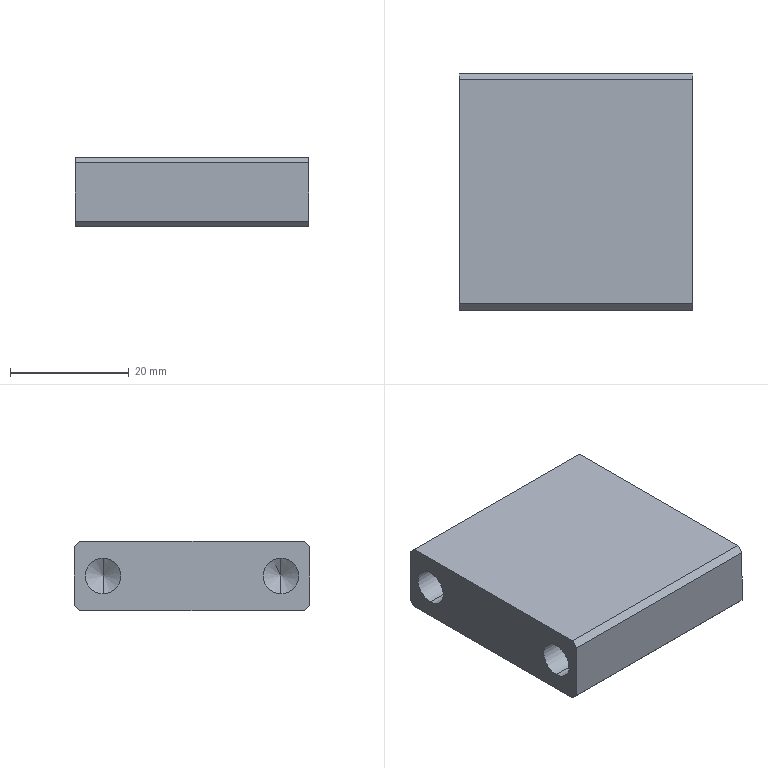Component | SolidWorks | ChainPartInnerSpacer-1 | 1 solid | 26 faces | box 39.4 x 39.8 x 11.8 mm | volume 16661 mm3 | plane 10 | cylinder 8 | cone 8 | commonest cylinder face diameters 6 x8
build123d program:
from build123d import *

# Parameters (mm, degrees)
SKETCH1_W             = 11.8
SKETCH1_H             = 39.8
BOSS_EXTRUDE1_DEPTH   = 19.7
M6_TAPPED_HOLE2_D     = 6
M6_TAPPED_HOLE2_DEPTH = 15
M6_TAPPED_HOLE2_TIP   = 1.803
M6_TAPPED_HOLE3_D     = 6
M6_TAPPED_HOLE3_DEPTH = 15
M6_TAPPED_HOLE3_TIP   = 1.803
CHAMFER1_SIZE         = 1


with BuildPart() as part:
    # Sketch1 → Boss-Extrude1 (new, symmetric)
    with BuildSketch(Plane.XY):
        Rectangle(SKETCH1_W, SKETCH1_H)
    extrude(amount=BOSS_EXTRUDE1_DEPTH, both=True)

    # M6 Tapped Hole2
    with Locations(Plane.XY.offset(19.7)):
        with Locations((0, 15), (0, -15)):
            Hole(M6_TAPPED_HOLE2_D / 2, depth=M6_TAPPED_HOLE2_DEPTH)
            with Locations((0, 0, -(M6_TAPPED_HOLE2_DEPTH + M6_TAPPED_HOLE2_TIP / 2))):  # 118° drill point
                Cone(0, M6_TAPPED_HOLE2_D / 2, M6_TAPPED_HOLE2_TIP, mode=Mode.SUBTRACT)

    # M6 Tapped Hole3
    with Locations(Plane(origin=(0, 0, -19.7), x_dir=(-1, 0, 0), z_dir=(0, 0, -1))):
        with Locations((0, 15), (0, -15)):
            Hole(M6_TAPPED_HOLE3_D / 2, depth=M6_TAPPED_HOLE3_DEPTH)
            with Locations((0, 0, -(M6_TAPPED_HOLE3_DEPTH + M6_TAPPED_HOLE3_TIP / 2))):  # 118° drill point
                Cone(0, M6_TAPPED_HOLE3_D / 2, M6_TAPPED_HOLE3_TIP, mode=Mode.SUBTRACT)

    # Chamfer1
    chamfer1_edges = [part.edges().sort_by_distance(p)[0] for p in [
        (-5.9, 19.9, 0),
        (5.9, 19.9, 0),
        (5.9, -19.9, 0),
        (-5.9, -19.9, 0),
    ]]
    chamfer(chamfer1_edges, length=CHAMFER1_SIZE)


solid = part.part

# Placed as in the assembly
solid = solid.moved(Location((107.937, -2.563, -115.304), (0, 90, 0)))